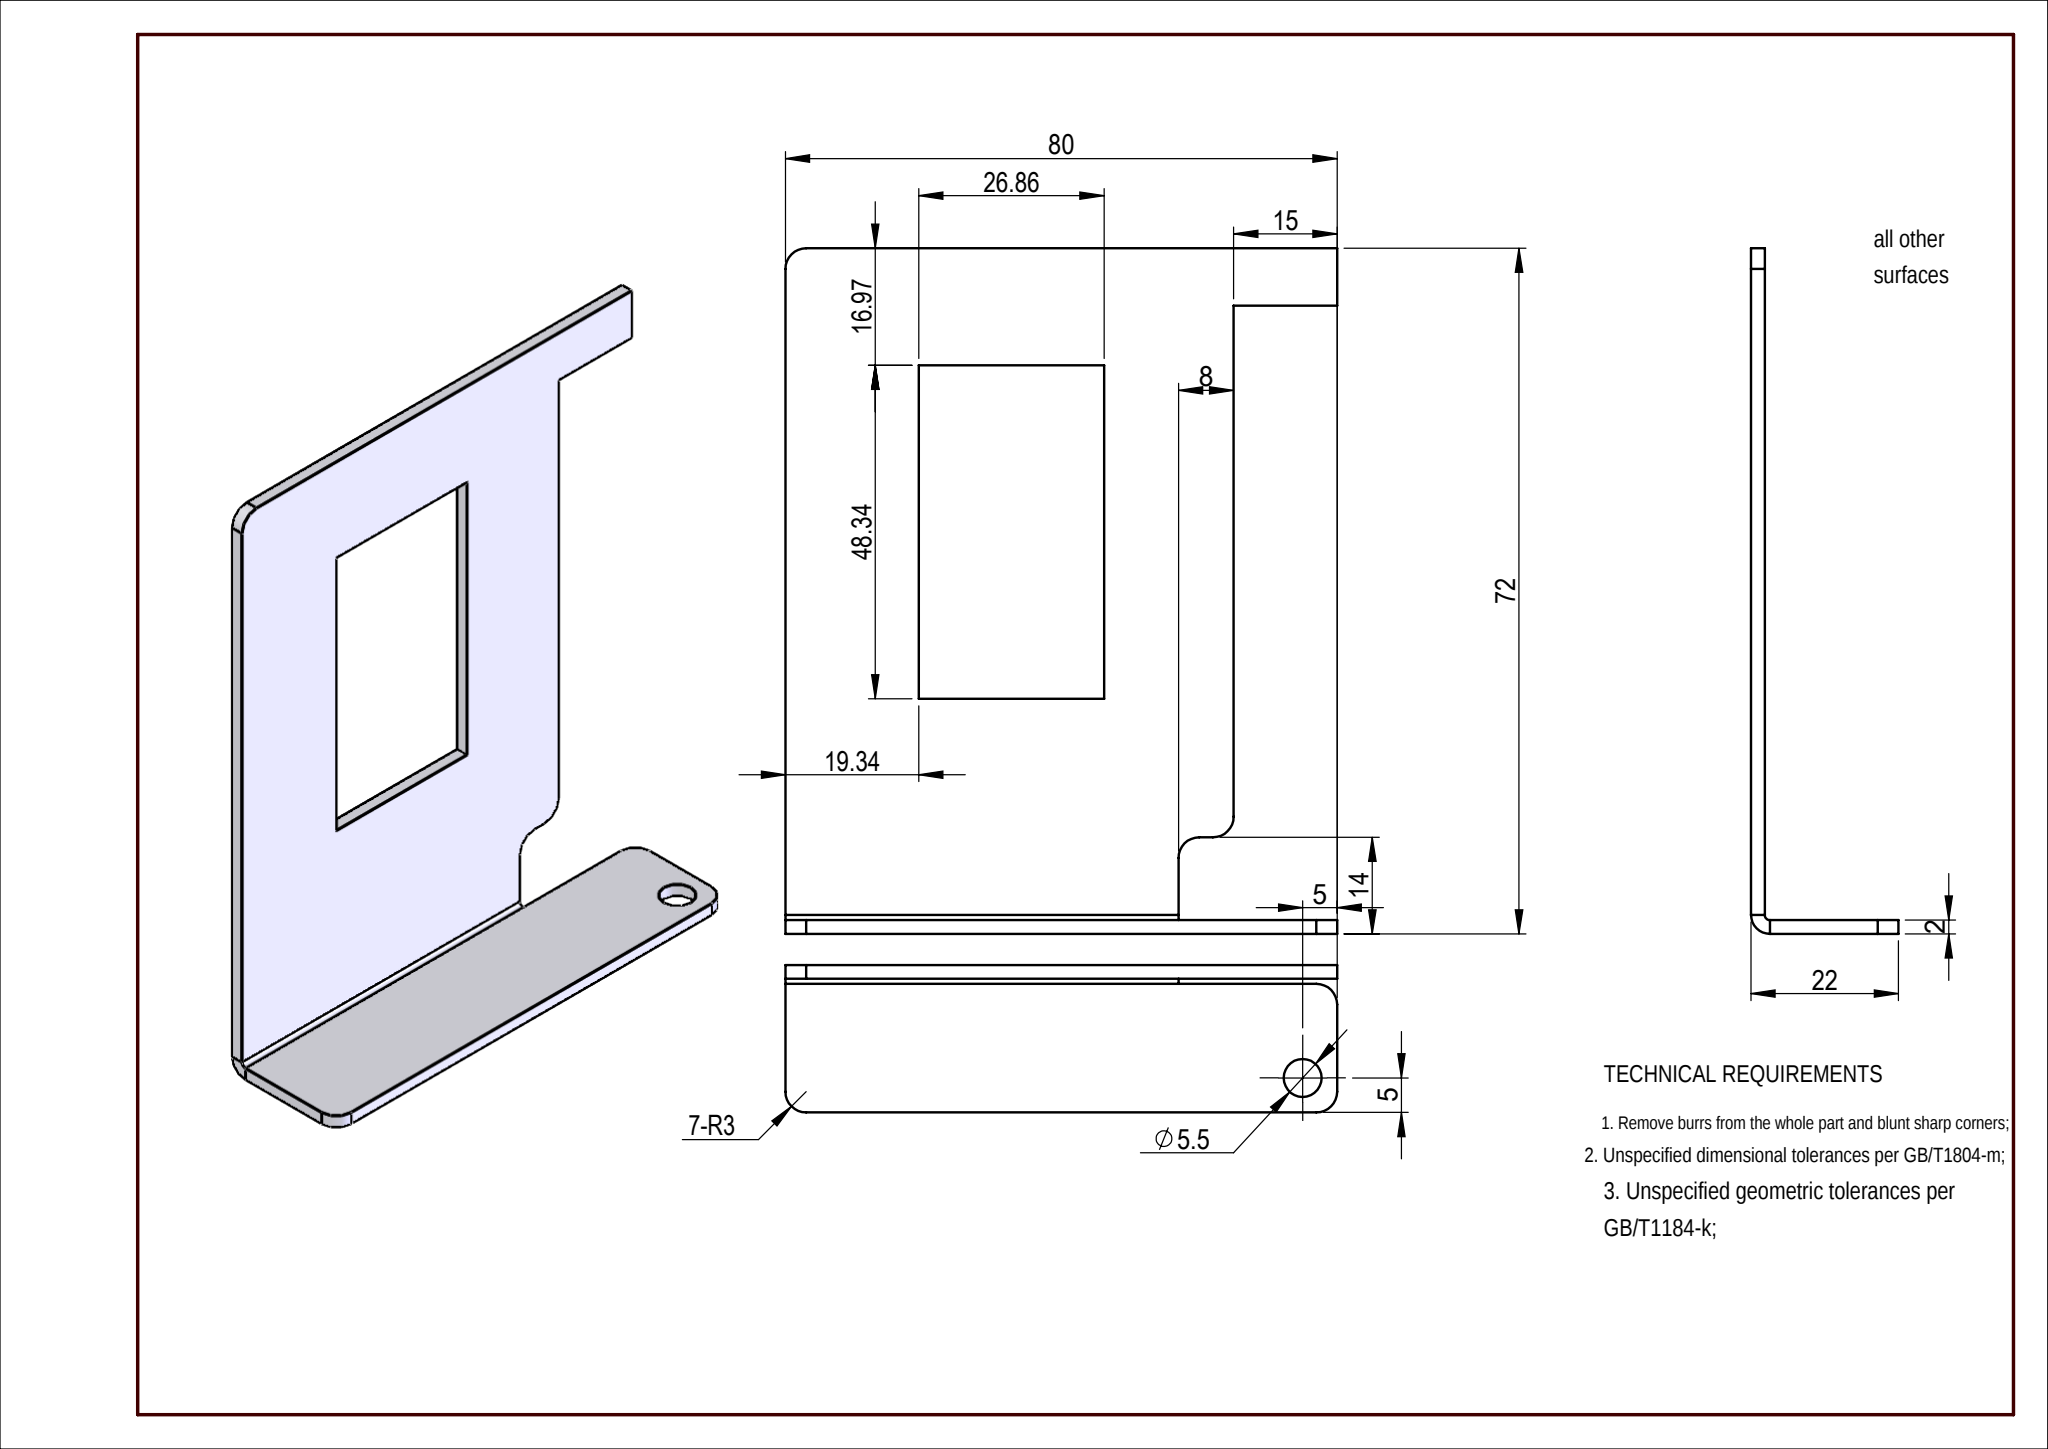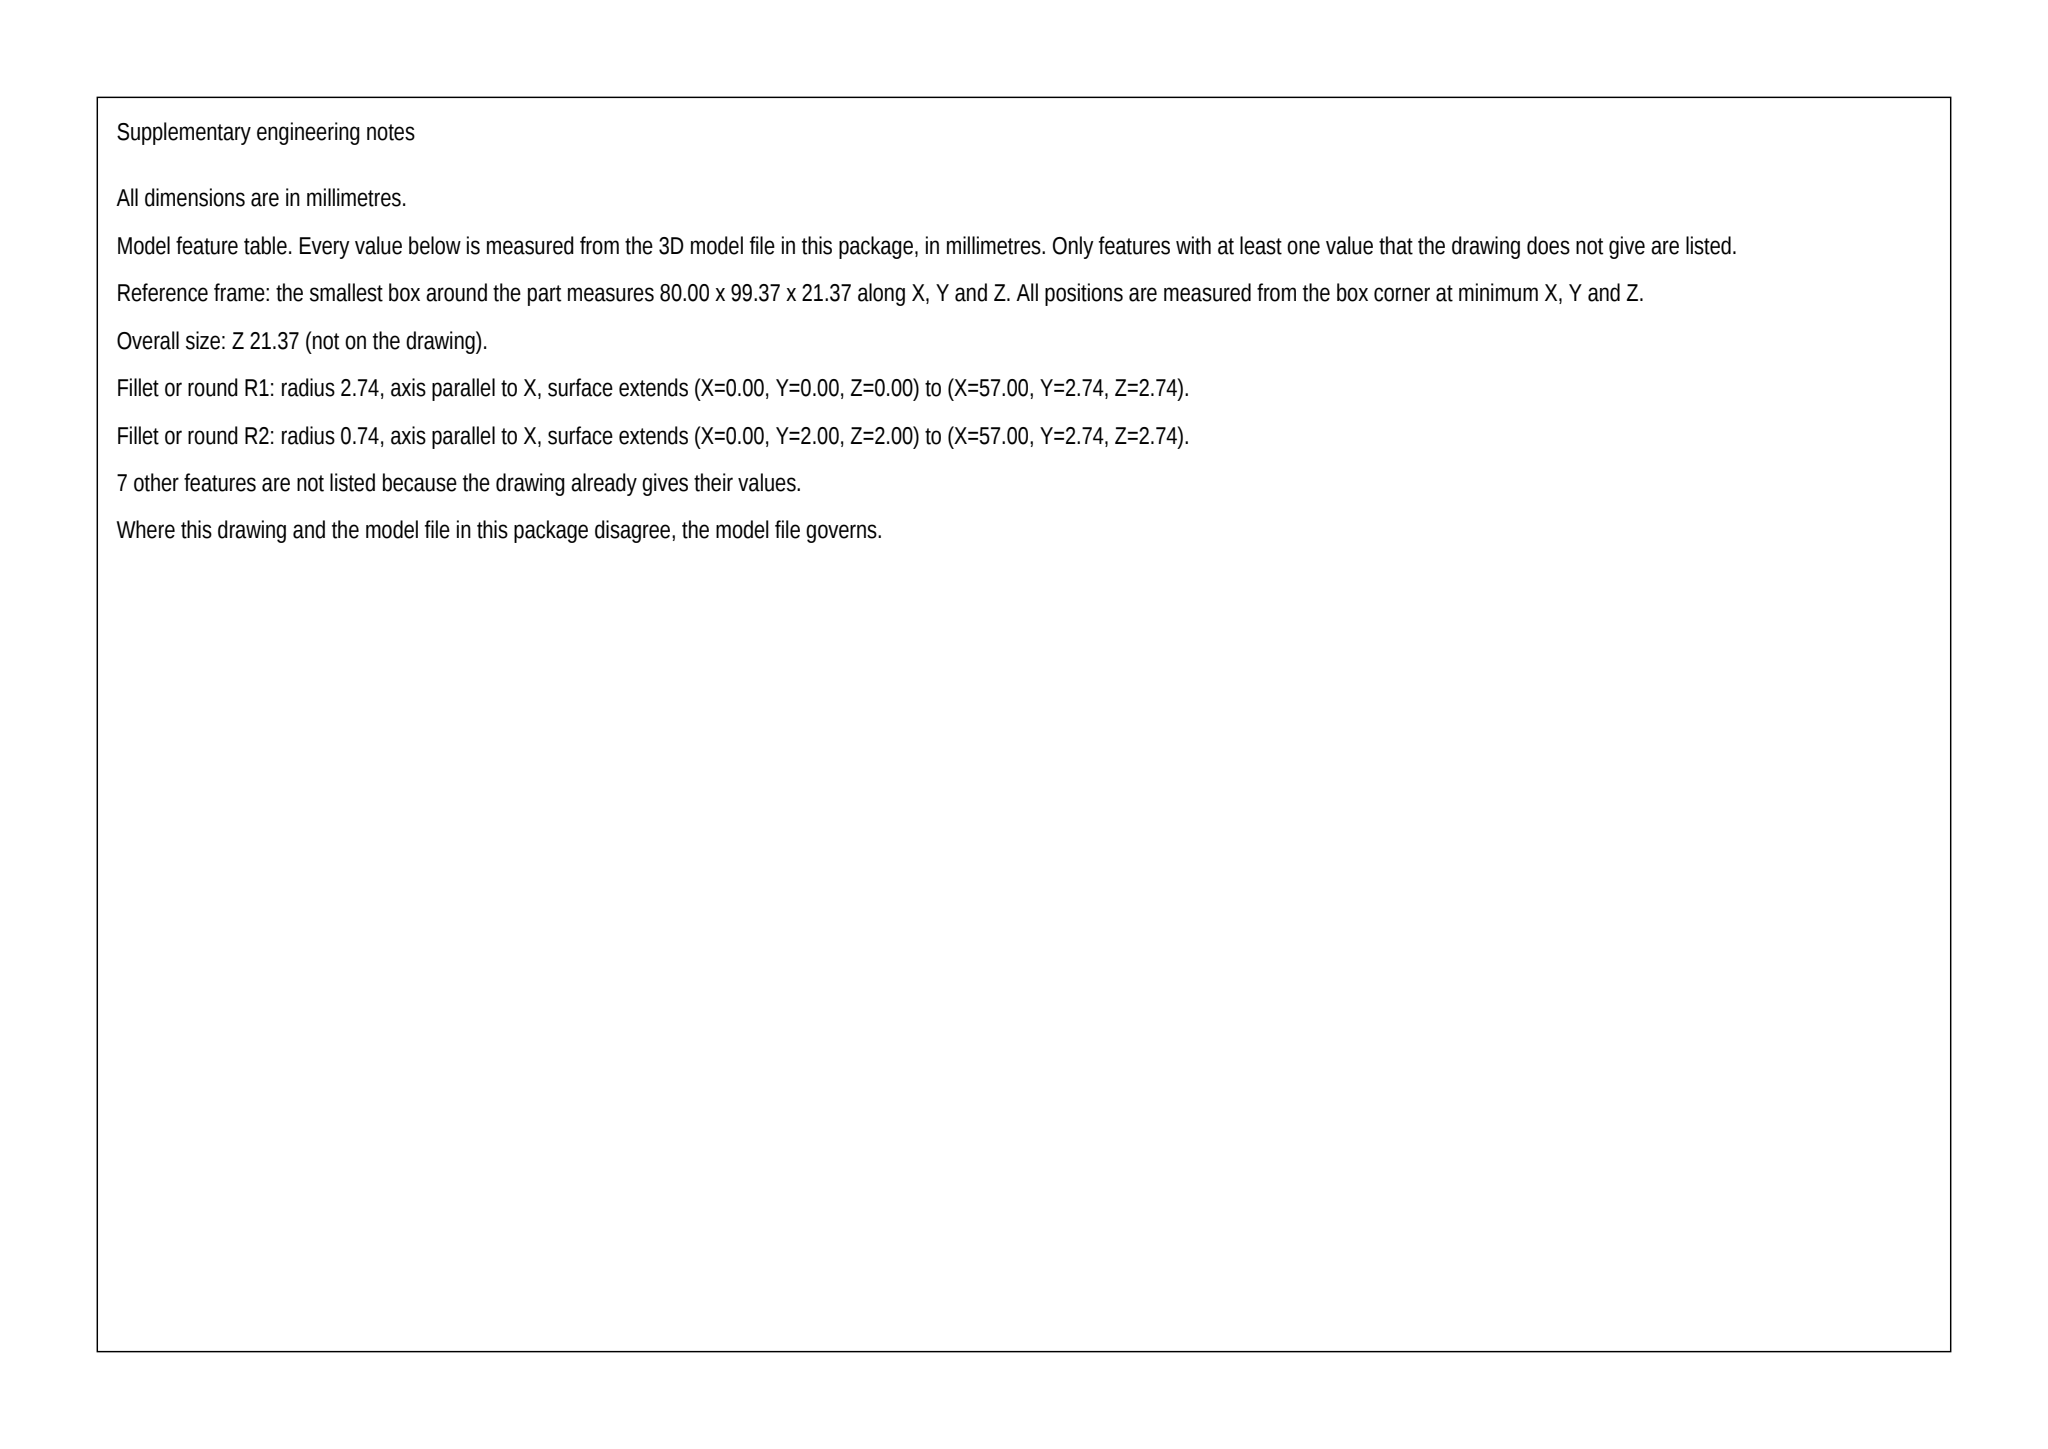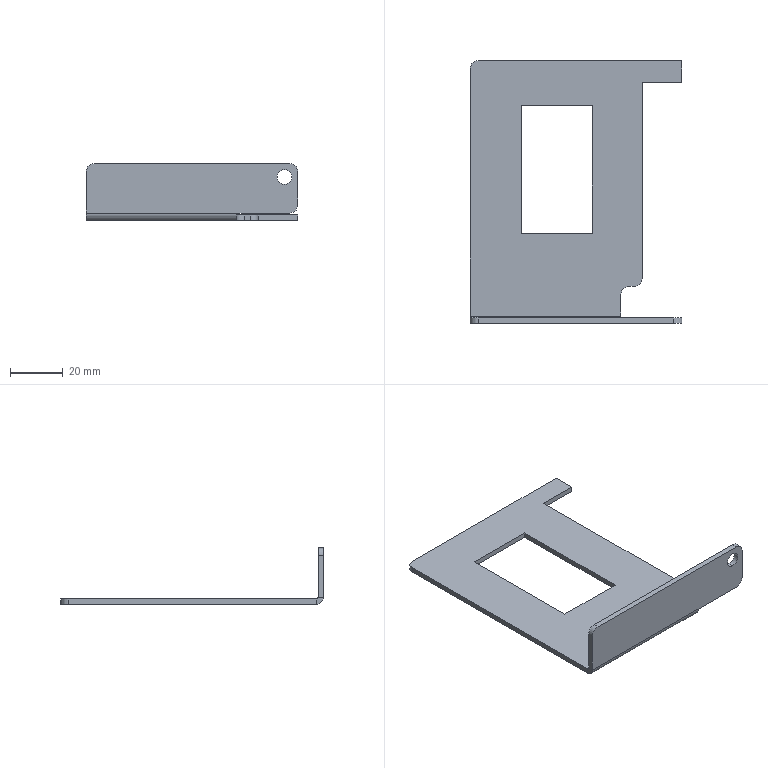Part | SolidWorks | mm | 1 solid | 31 faces | box 80 x 99.37 x 21.37 mm | volume 13265 mm3 | plane 21 | cylinder 10 | commonest cylinder face diameters 6 x6 5.5 x2 5.473 x1 1.473 x1